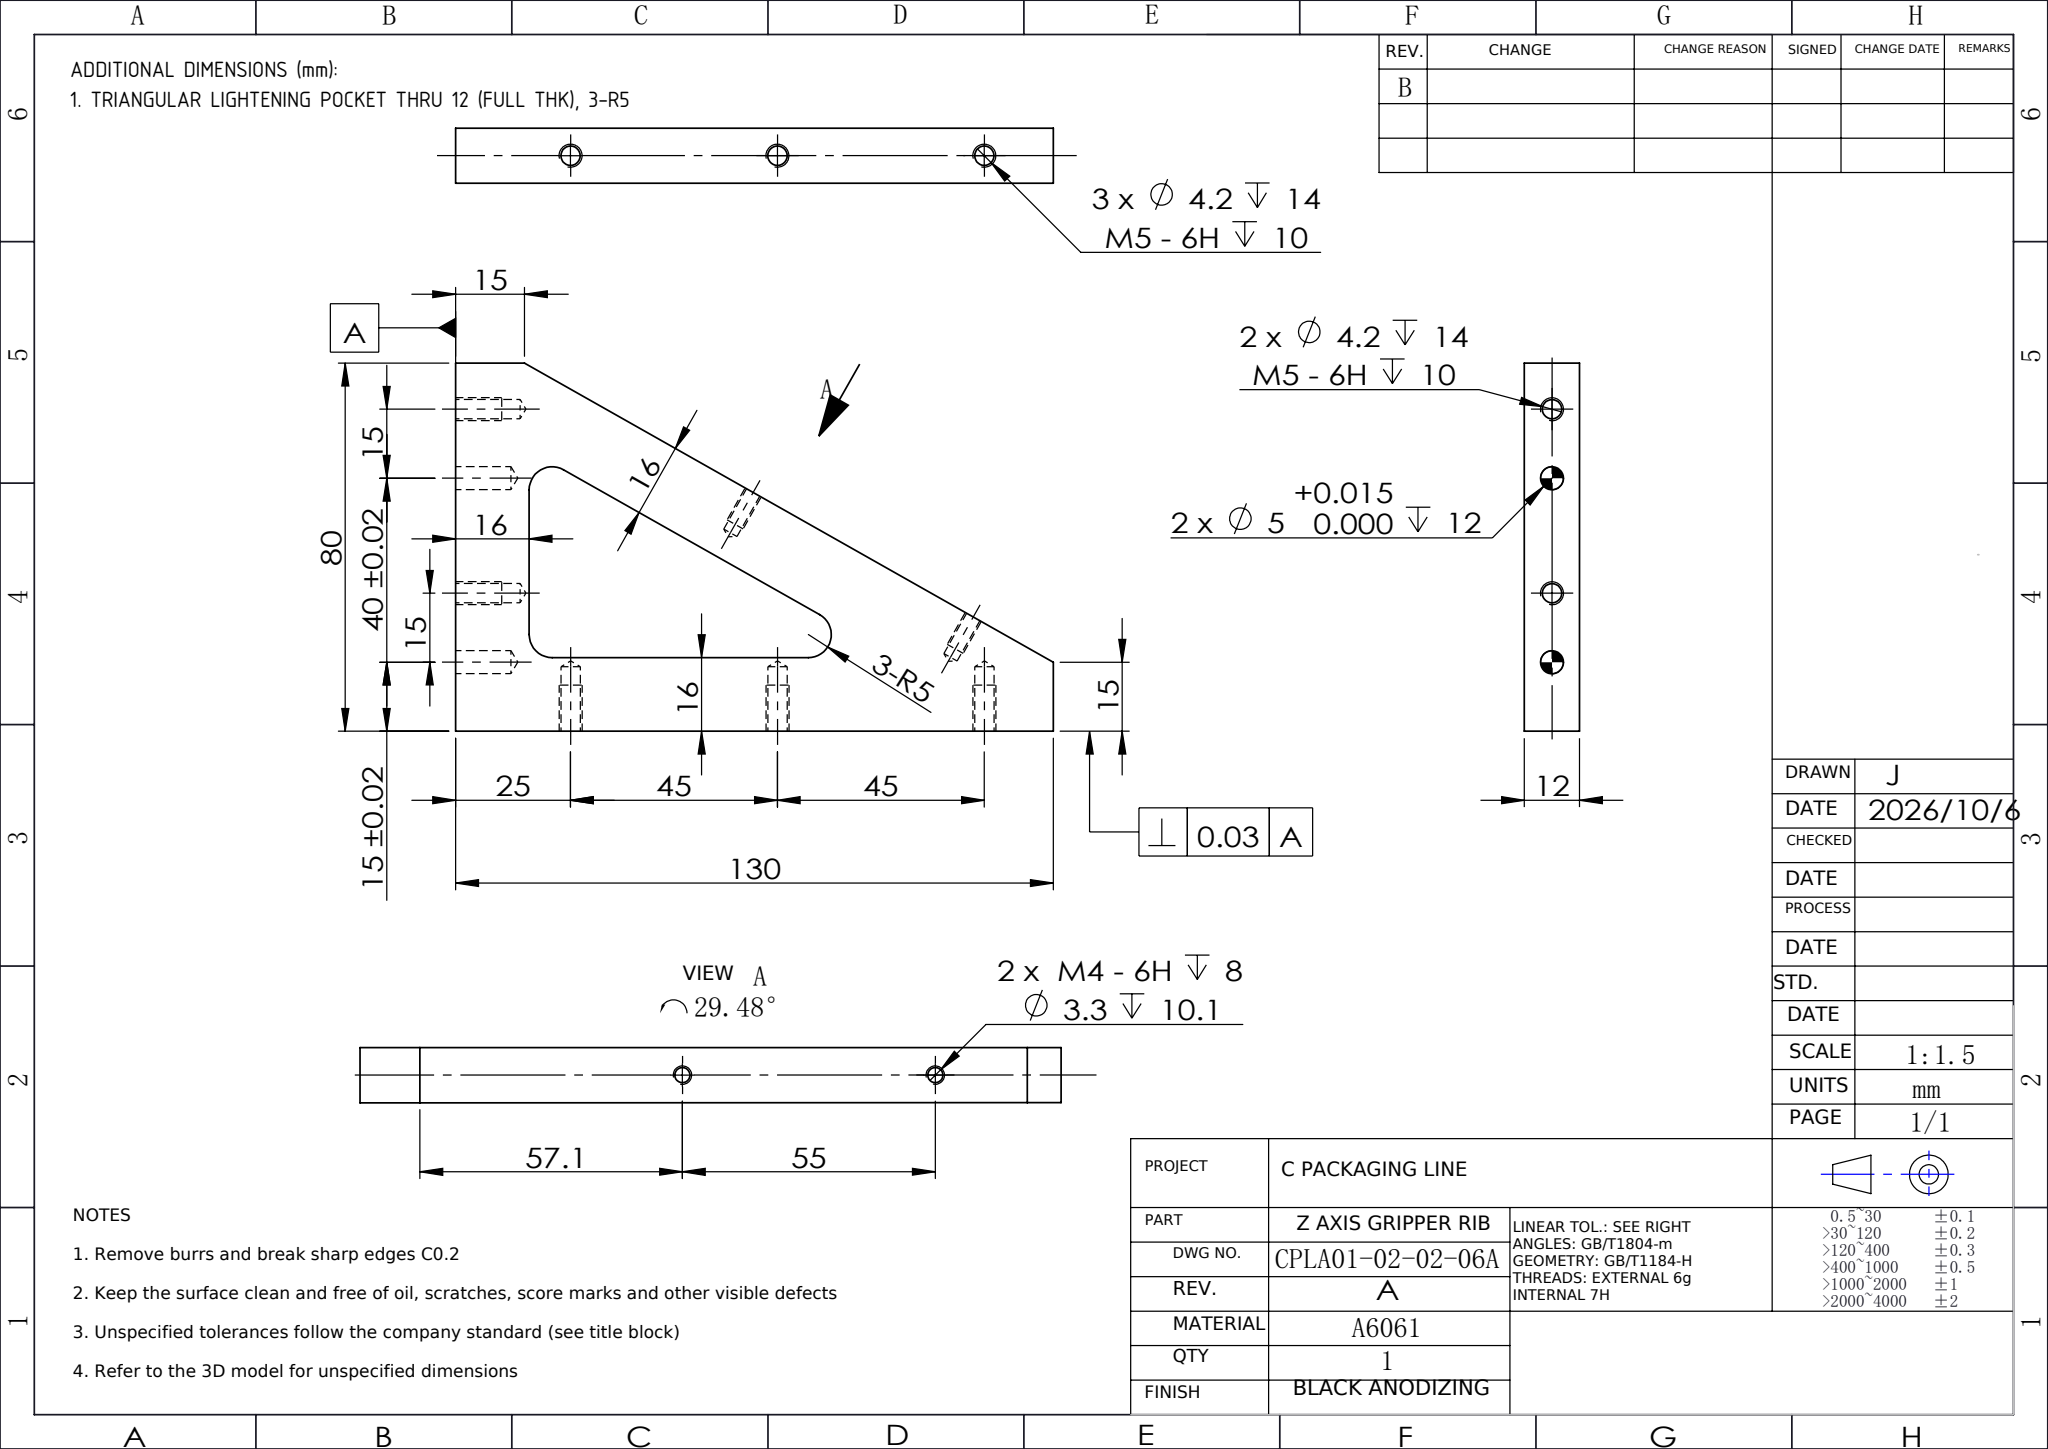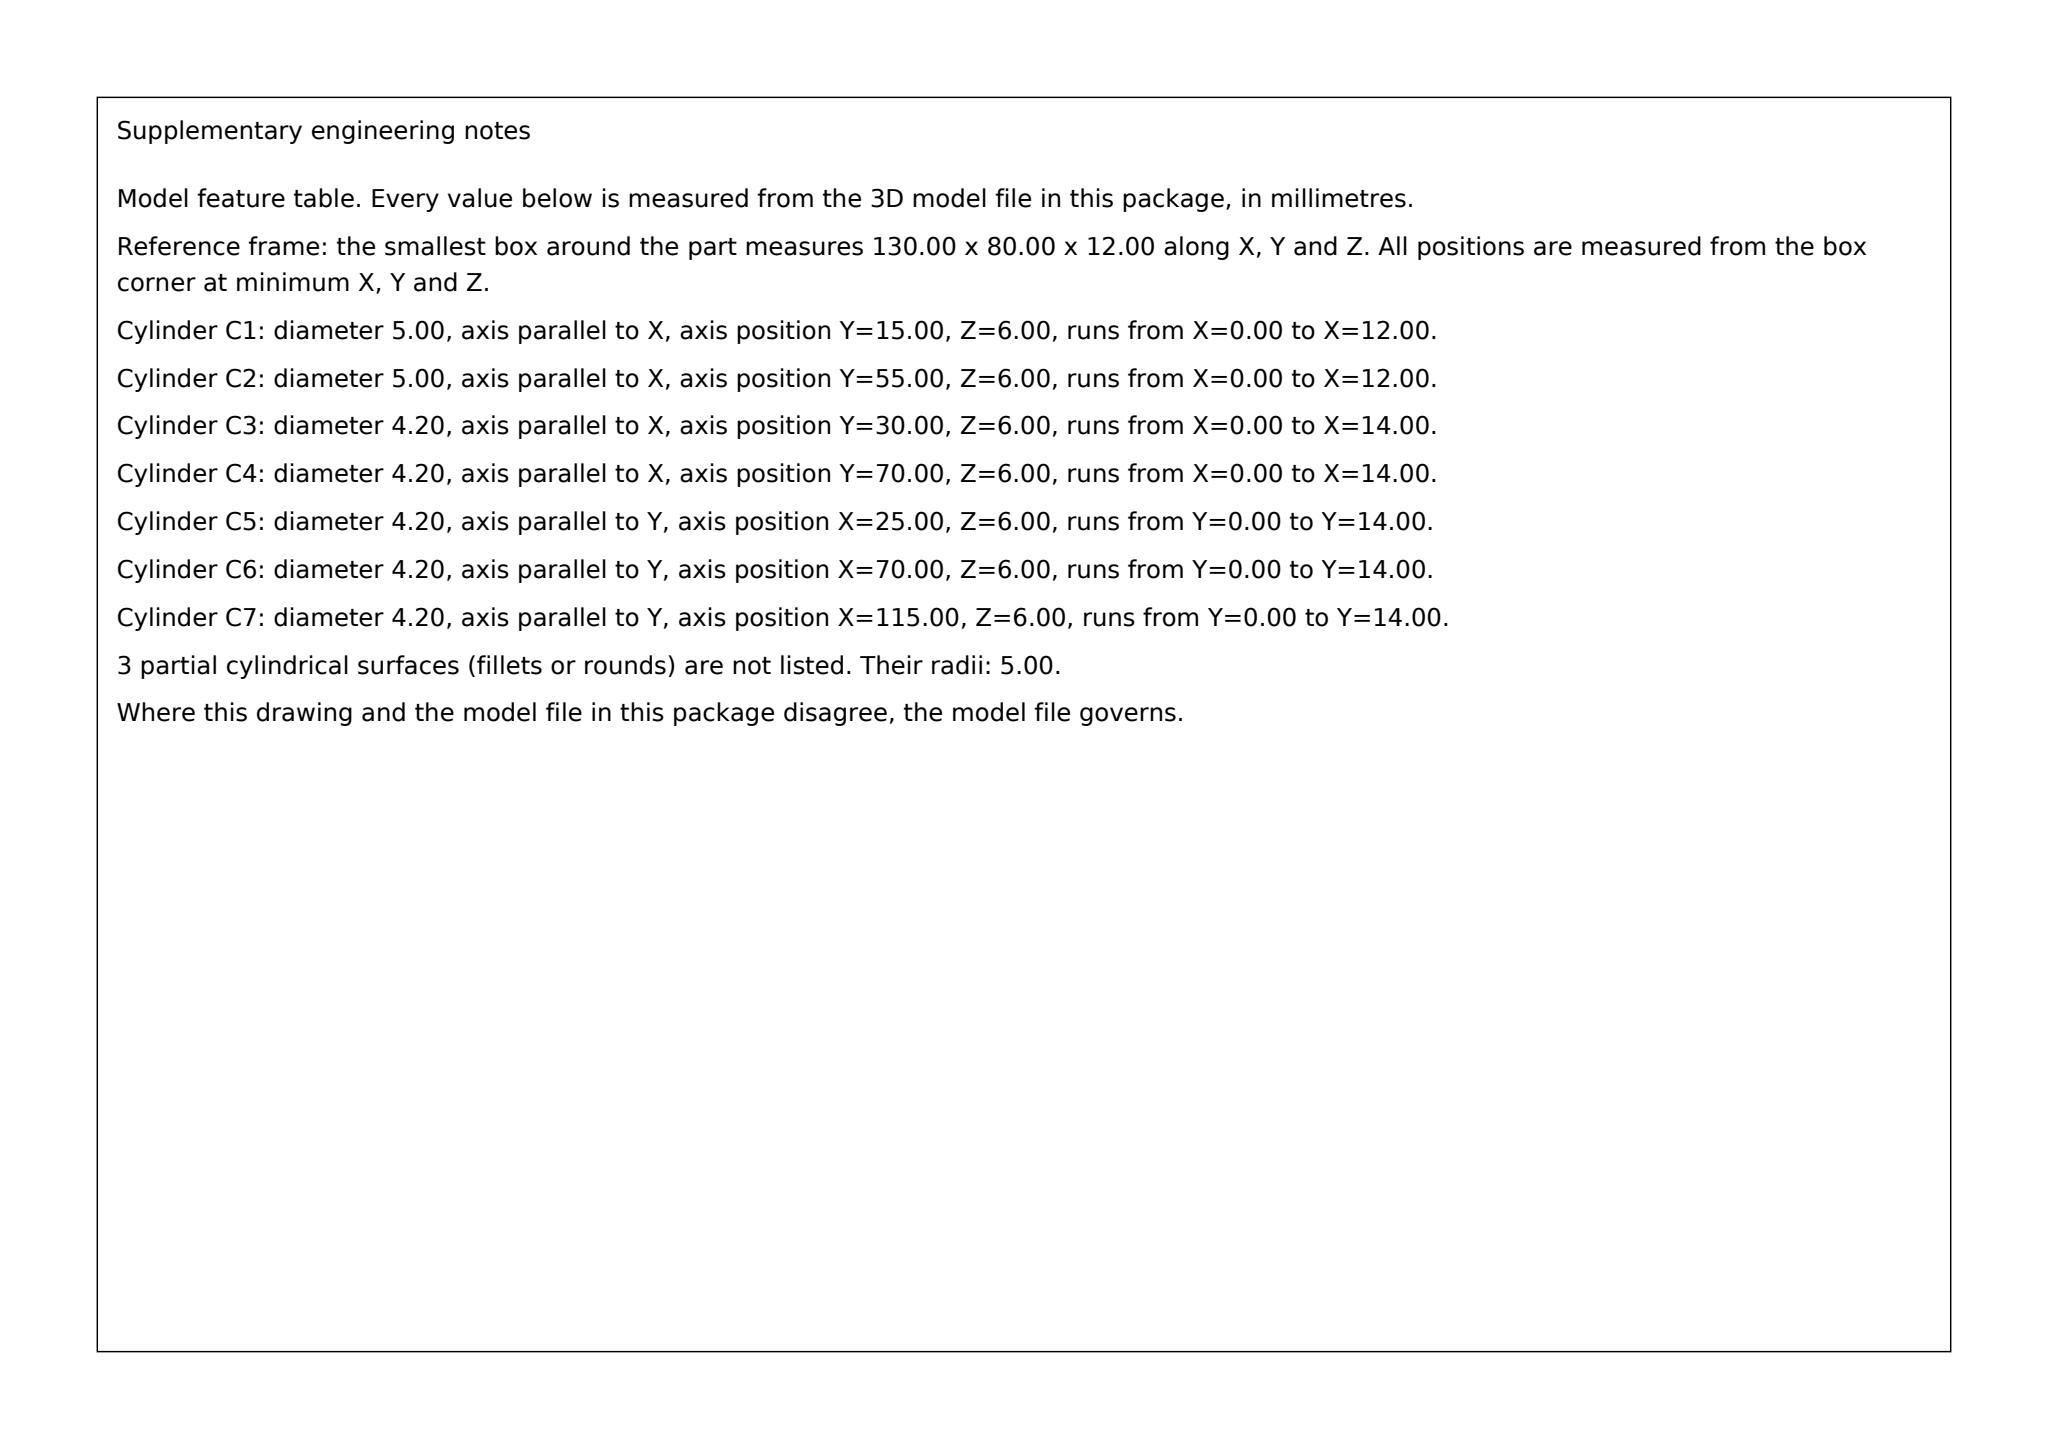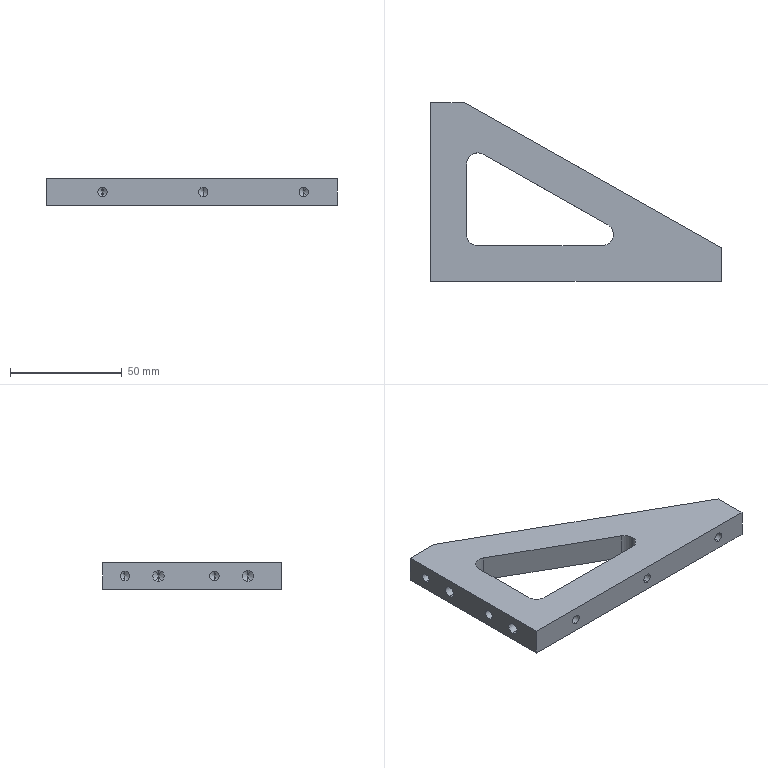Part | SolidWorks | mm | 1 solid | 50 faces | box 130 x 80 x 12 mm | volume 57744 mm3 | cylinder 22 | cone 18 | plane 10 | commonest cylinder face diameters 4.2 x10 5 x4 3.3 x4 10 x4
build123d program:
from build123d import *

# Parameters (mm, degrees)
BOSS_EXTRUDE1_DEPTH           = 6
M5_TAPPED_HOLE2_D             = 4.2
M5_TAPPED_HOLE2_DEPTH         = 14
M5_TAPPED_HOLE2_TIP           = 1.262
M5_TAPPED_HOLE3_D             = 4.2
M5_TAPPED_HOLE3_DEPTH         = 14
M5_TAPPED_HOLE3_TIP           = 1.262
CUT_EXTRUDE1_DEPTH            = 154.114
FILLET1_R                     = 5
M4_TAPPED_HOLE1_D             = 3.3
M4_TAPPED_HOLE1_DEPTH         = 10.1
M4_TAPPED_HOLE1_TIP           = 0.9914
F_5_0MM_DOWEL_PIN_HOLE1_D     = 5
F_5_0MM_DOWEL_PIN_HOLE1_DEPTH = 12
F_5_0MM_DOWEL_PIN_HOLE1_TIP   = 1.502


with BuildPart() as part:
    # Sketch2 → Boss-Extrude1 (new, symmetric)
    with BuildSketch(Plane.XY):
        Polygon((0, 0), (130, 0), (130, 15), (15, 80), (0, 80), align=None)
    extrude(amount=BOSS_EXTRUDE1_DEPTH, both=True)

    # M5 Tapped Hole2
    with Locations(Plane(origin=(0, 0, 0), x_dir=(-1, 0, 0), z_dir=(0, -1, 0))):
        with Locations((-25, 0), (-70, 0), (-115, 0)):
            Hole(M5_TAPPED_HOLE2_D / 2, depth=M5_TAPPED_HOLE2_DEPTH)
            with Locations((0, 0, -(M5_TAPPED_HOLE2_DEPTH + M5_TAPPED_HOLE2_TIP / 2))):  # 118° drill point
                Cone(0, M5_TAPPED_HOLE2_D / 2, M5_TAPPED_HOLE2_TIP, mode=Mode.SUBTRACT)

    # M5 Tapped Hole3
    with Locations(Plane.ZY):
        with Locations((0, 30), (0, 70)):
            Hole(M5_TAPPED_HOLE3_D / 2, depth=M5_TAPPED_HOLE3_DEPTH)
            with Locations((0, 0, -(M5_TAPPED_HOLE3_DEPTH + M5_TAPPED_HOLE3_TIP / 2))):  # 118° drill point
                Cone(0, M5_TAPPED_HOLE3_D / 2, M5_TAPPED_HOLE3_TIP, mode=Mode.SUBTRACT)

    # Sketch7 → Cut-Extrude1 (cut, through all)
    with BuildSketch(Plane(origin=(0, 0, -6), x_dir=(-1, 0, 0), z_dir=(0, 0, -1))):
        Polygon((-95.714, 16), (-16, 61.056), (-16, 16), align=None)
    extrude(amount=-CUT_EXTRUDE1_DEPTH, mode=Mode.SUBTRACT)

    # Fillet1
    fillet1_edges = [part.edges().sort_by_distance(p)[0] for p in [
        (16, 16, 0),
        (95.714, 16, 0),
        (16, 61.056, 0),
    ]]
    fillet(fillet1_edges, radius=FILLET1_R)

    # M4 Tapped Hole1
    with Locations(Plane(origin=(37.901, 67.056, 0), x_dir=(0.8706, -0.4921, 0), z_dir=(0.4921, 0.8706, 0))):
        with Locations((85.792, 0), (30.792, 0)):
            Hole(M4_TAPPED_HOLE1_D / 2, depth=M4_TAPPED_HOLE1_DEPTH)
            with Locations((0, 0, -(M4_TAPPED_HOLE1_DEPTH + M4_TAPPED_HOLE1_TIP / 2))):  # 118° drill point
                Cone(0, M4_TAPPED_HOLE1_D / 2, M4_TAPPED_HOLE1_TIP, mode=Mode.SUBTRACT)

    # 5.0mm Dowel Pin Hole1
    with Locations(Plane.ZY):
        with Locations((0, 55), (0, 15)):
            Hole(F_5_0MM_DOWEL_PIN_HOLE1_D / 2, depth=F_5_0MM_DOWEL_PIN_HOLE1_DEPTH)
            with Locations((0, 0, -(F_5_0MM_DOWEL_PIN_HOLE1_DEPTH + F_5_0MM_DOWEL_PIN_HOLE1_TIP / 2))):  # 118° drill point
                Cone(0, F_5_0MM_DOWEL_PIN_HOLE1_D / 2, F_5_0MM_DOWEL_PIN_HOLE1_TIP, mode=Mode.SUBTRACT)


solid = part.part